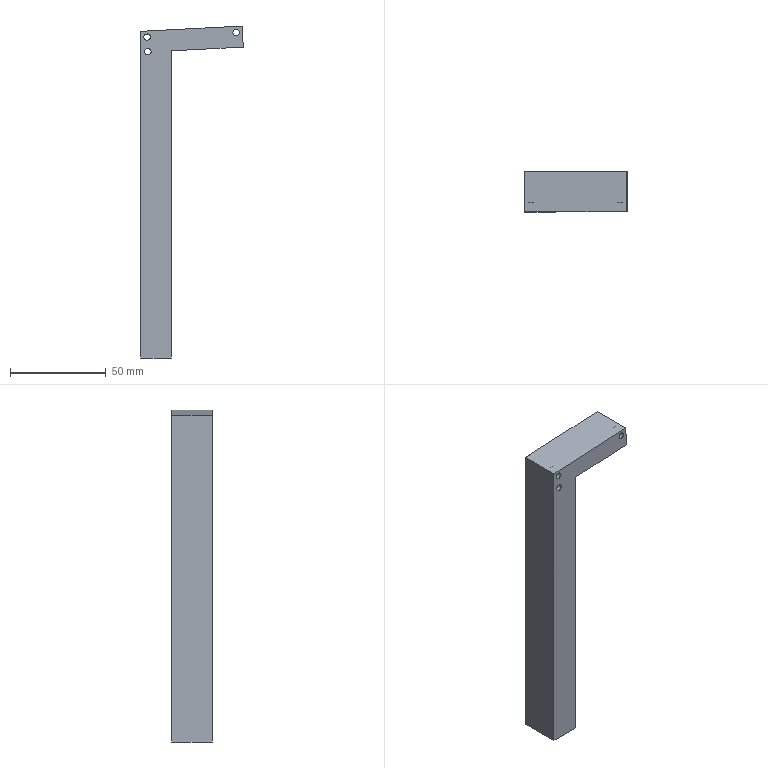Component | NX | SUPPORT_ROD | 1 solid | 17 faces | volume 64515 mm3 | plane 11 | cylinder 6 | commonest cylinder face diameters 3.3 x3 6 x3